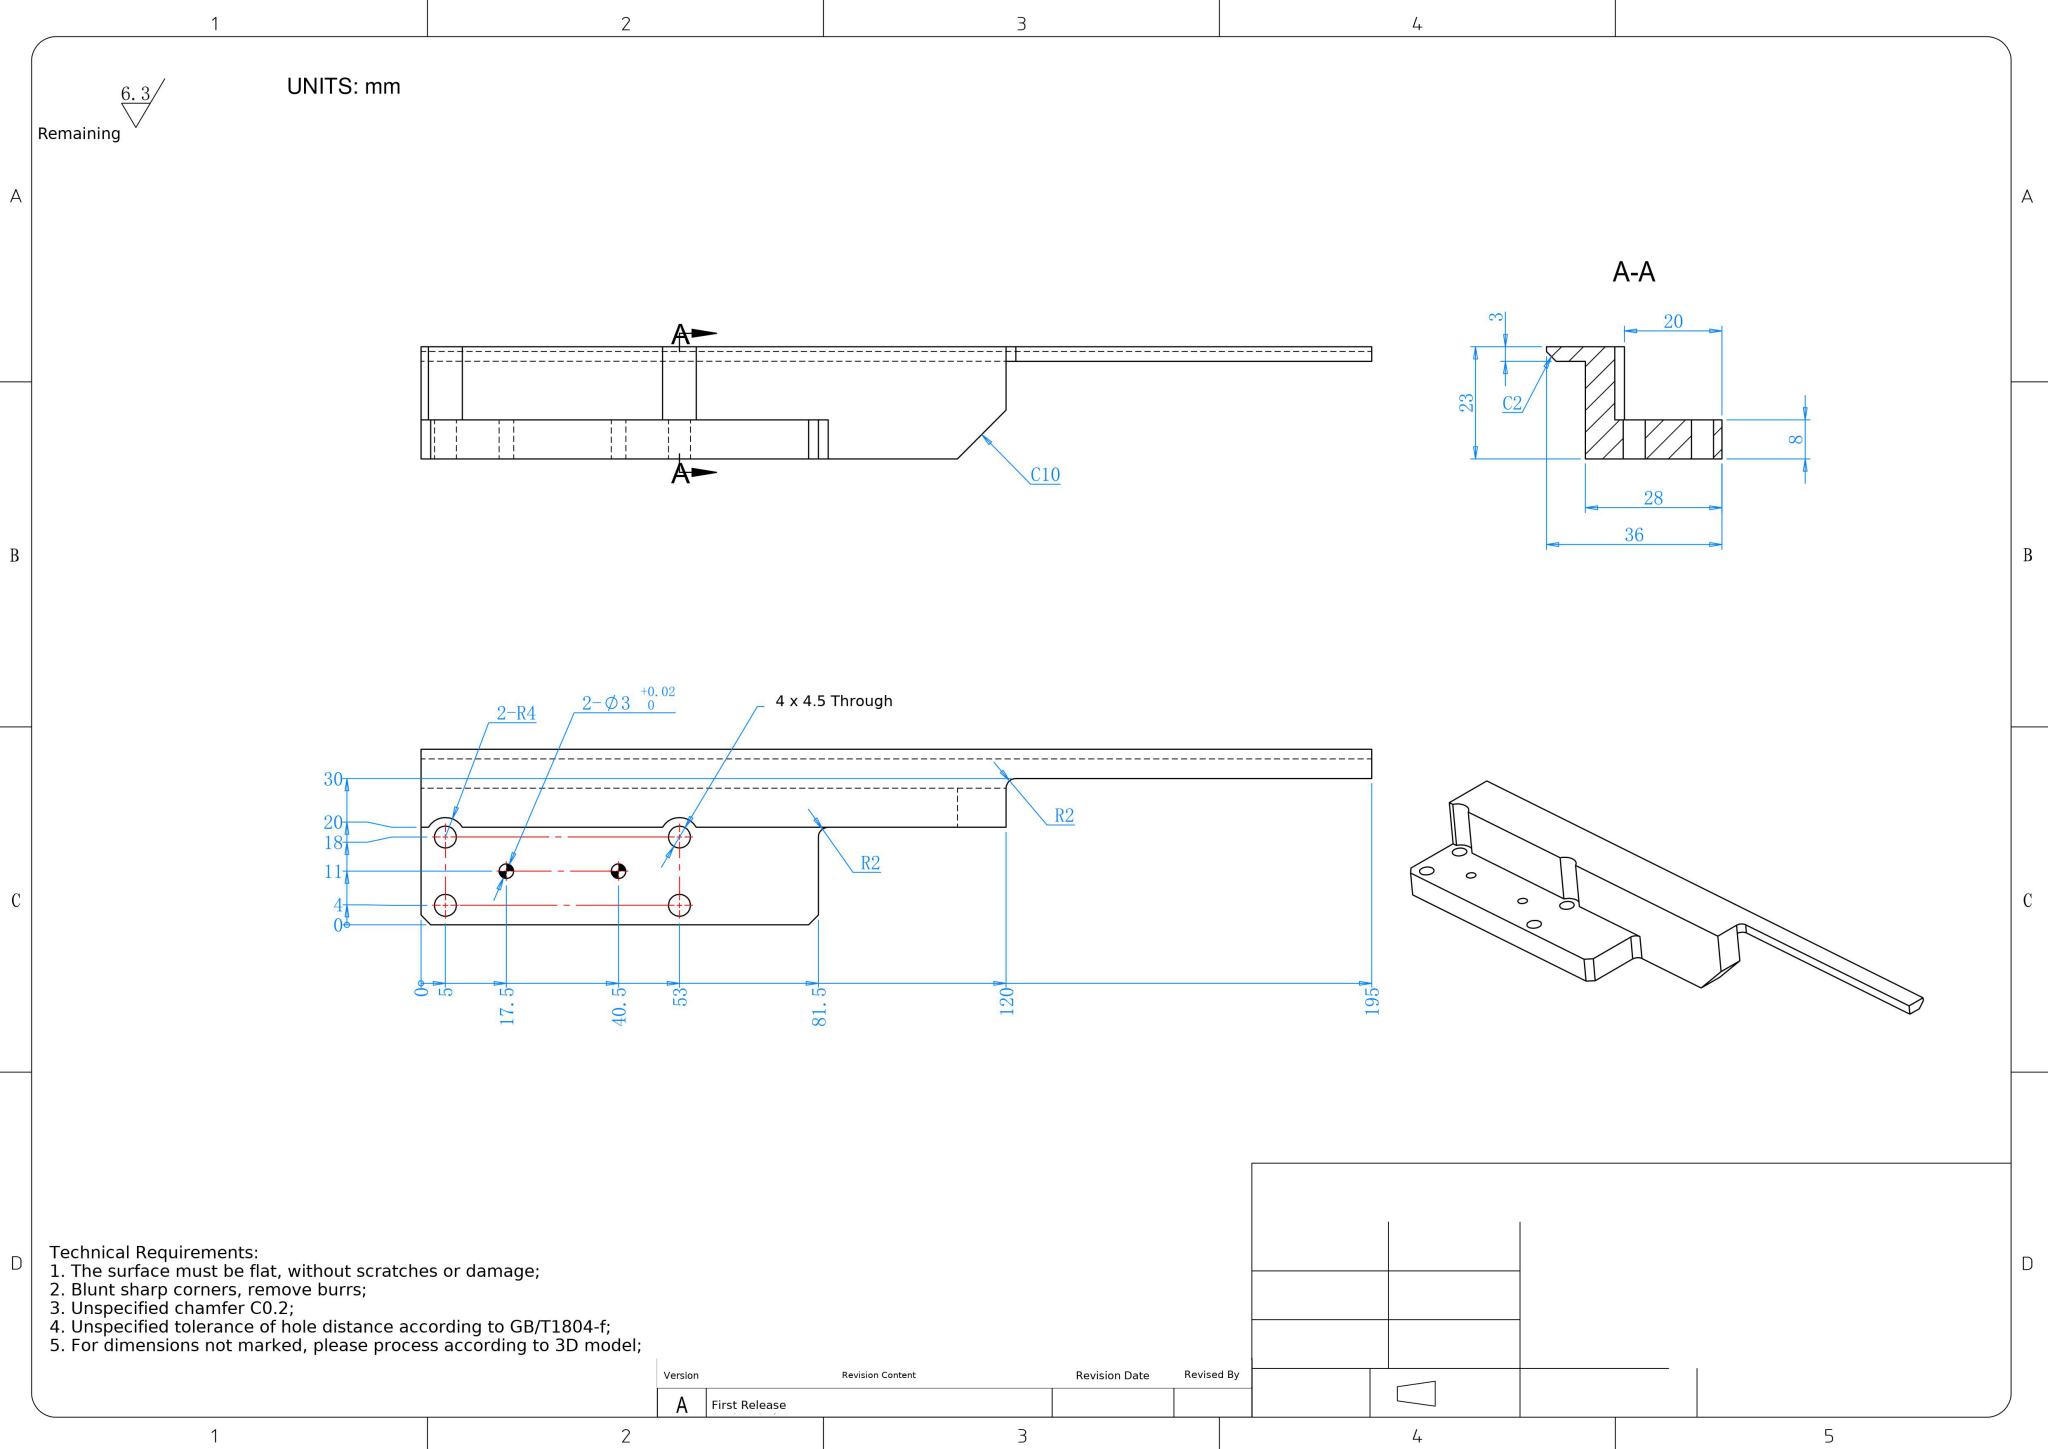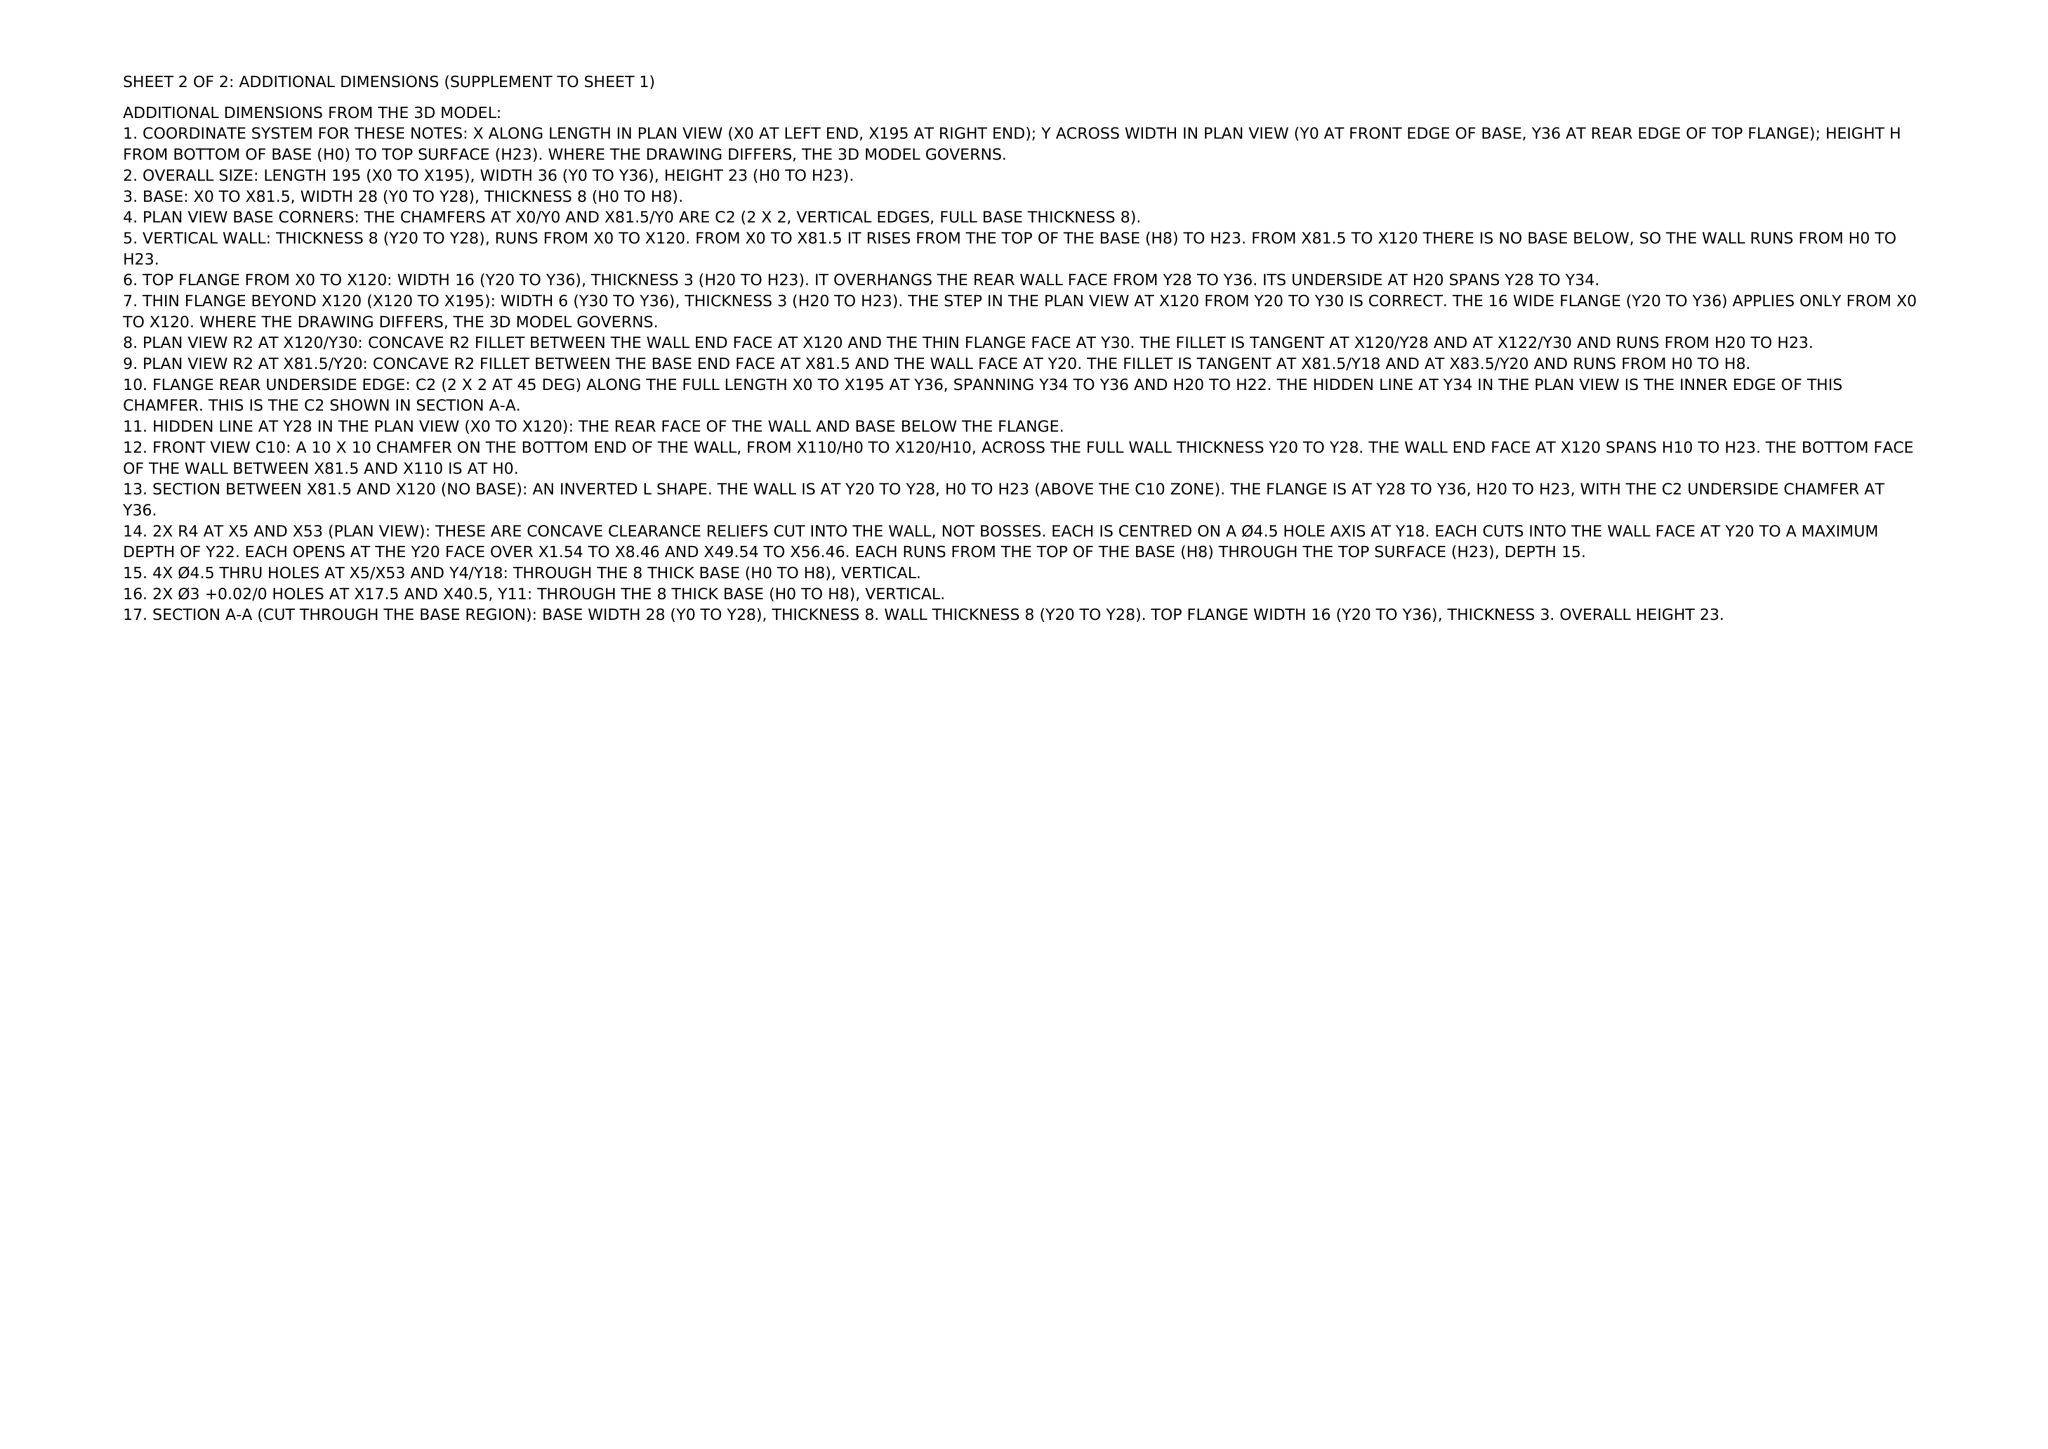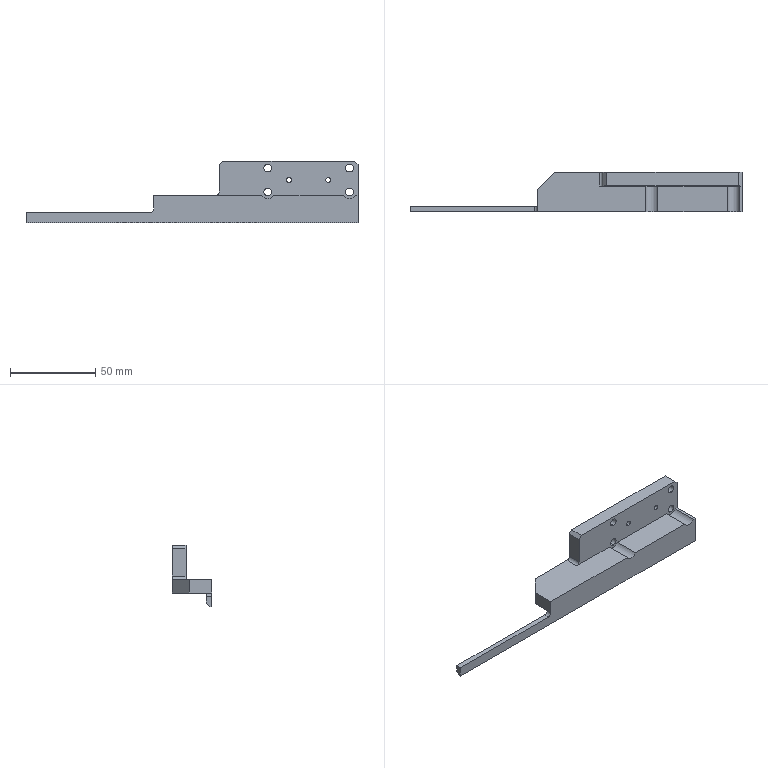Part | NX | mm | 1 solid | 35 faces | box 195 x 23 x 36 mm | volume 37621 mm3 | plane 19 | cylinder 16 | commonest cylinder face diameters 4.5 x8 3 x4 8 x2 4 x2